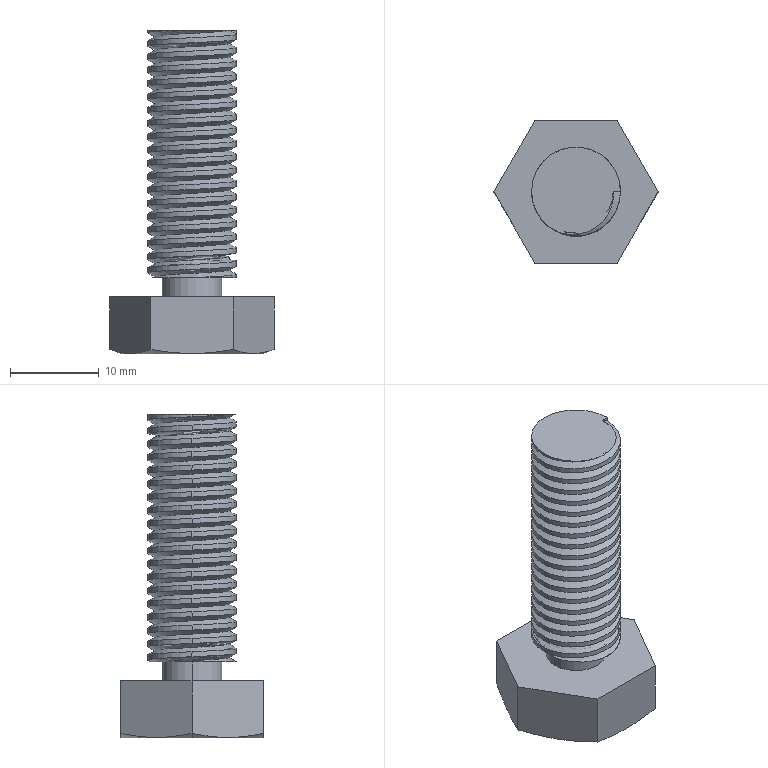Component | SolidWorks | M10-30Bolt1-1 | 1 solid | 56 faces | volume 3471 mm3 | cylinder 41 | plane 11 | cone 2 | spline 2 | commonest cylinder face diameters 10 x39 6.708 x2